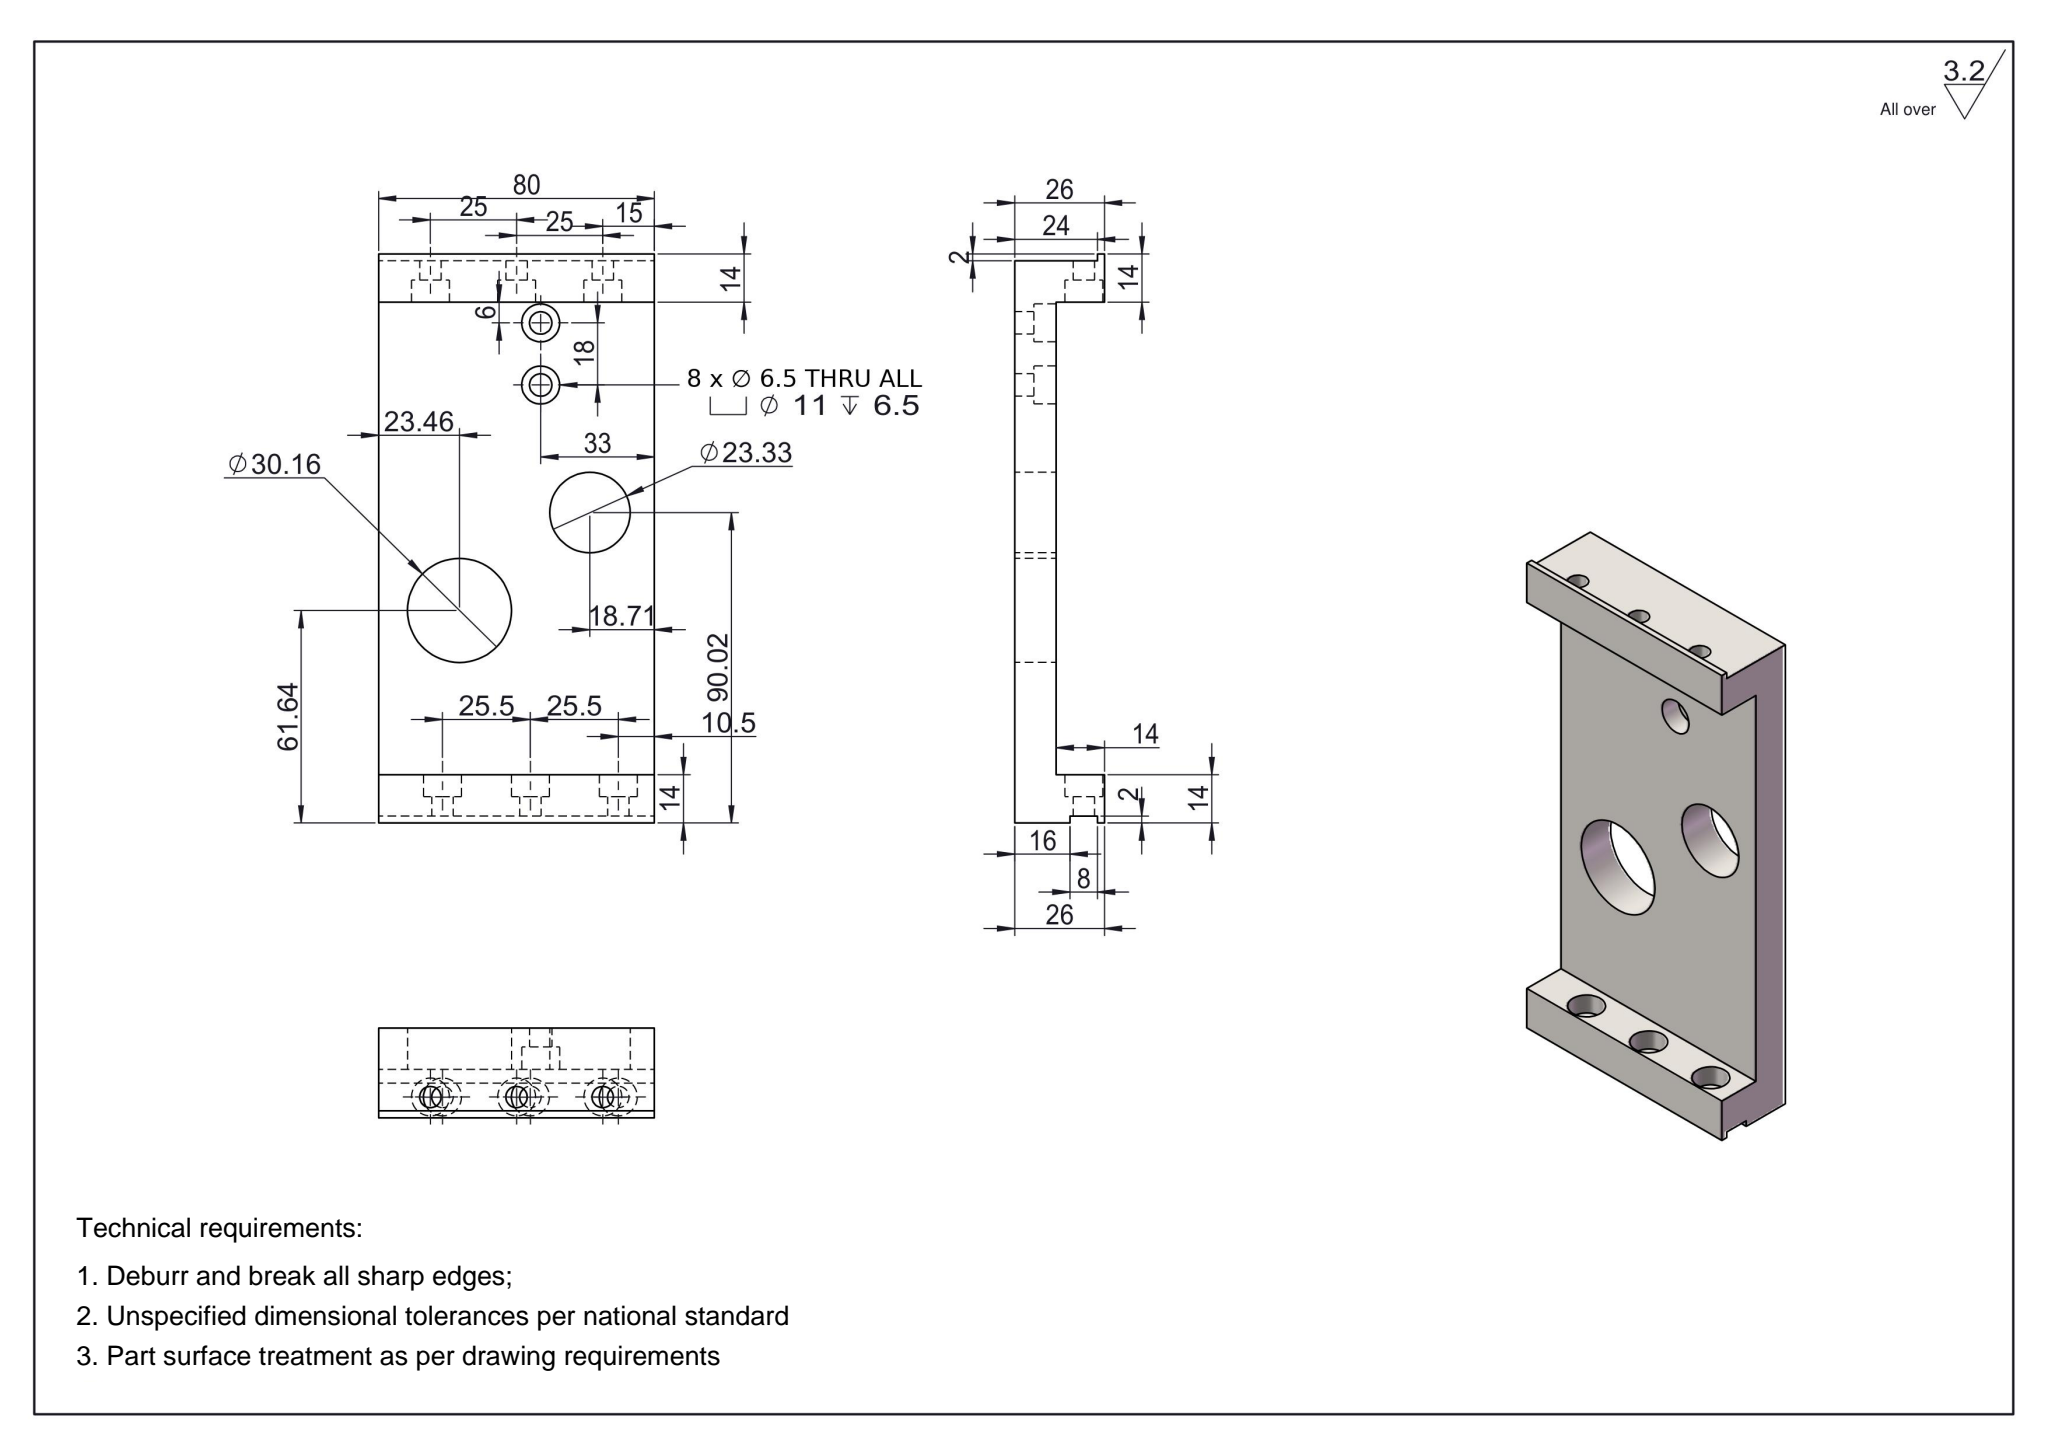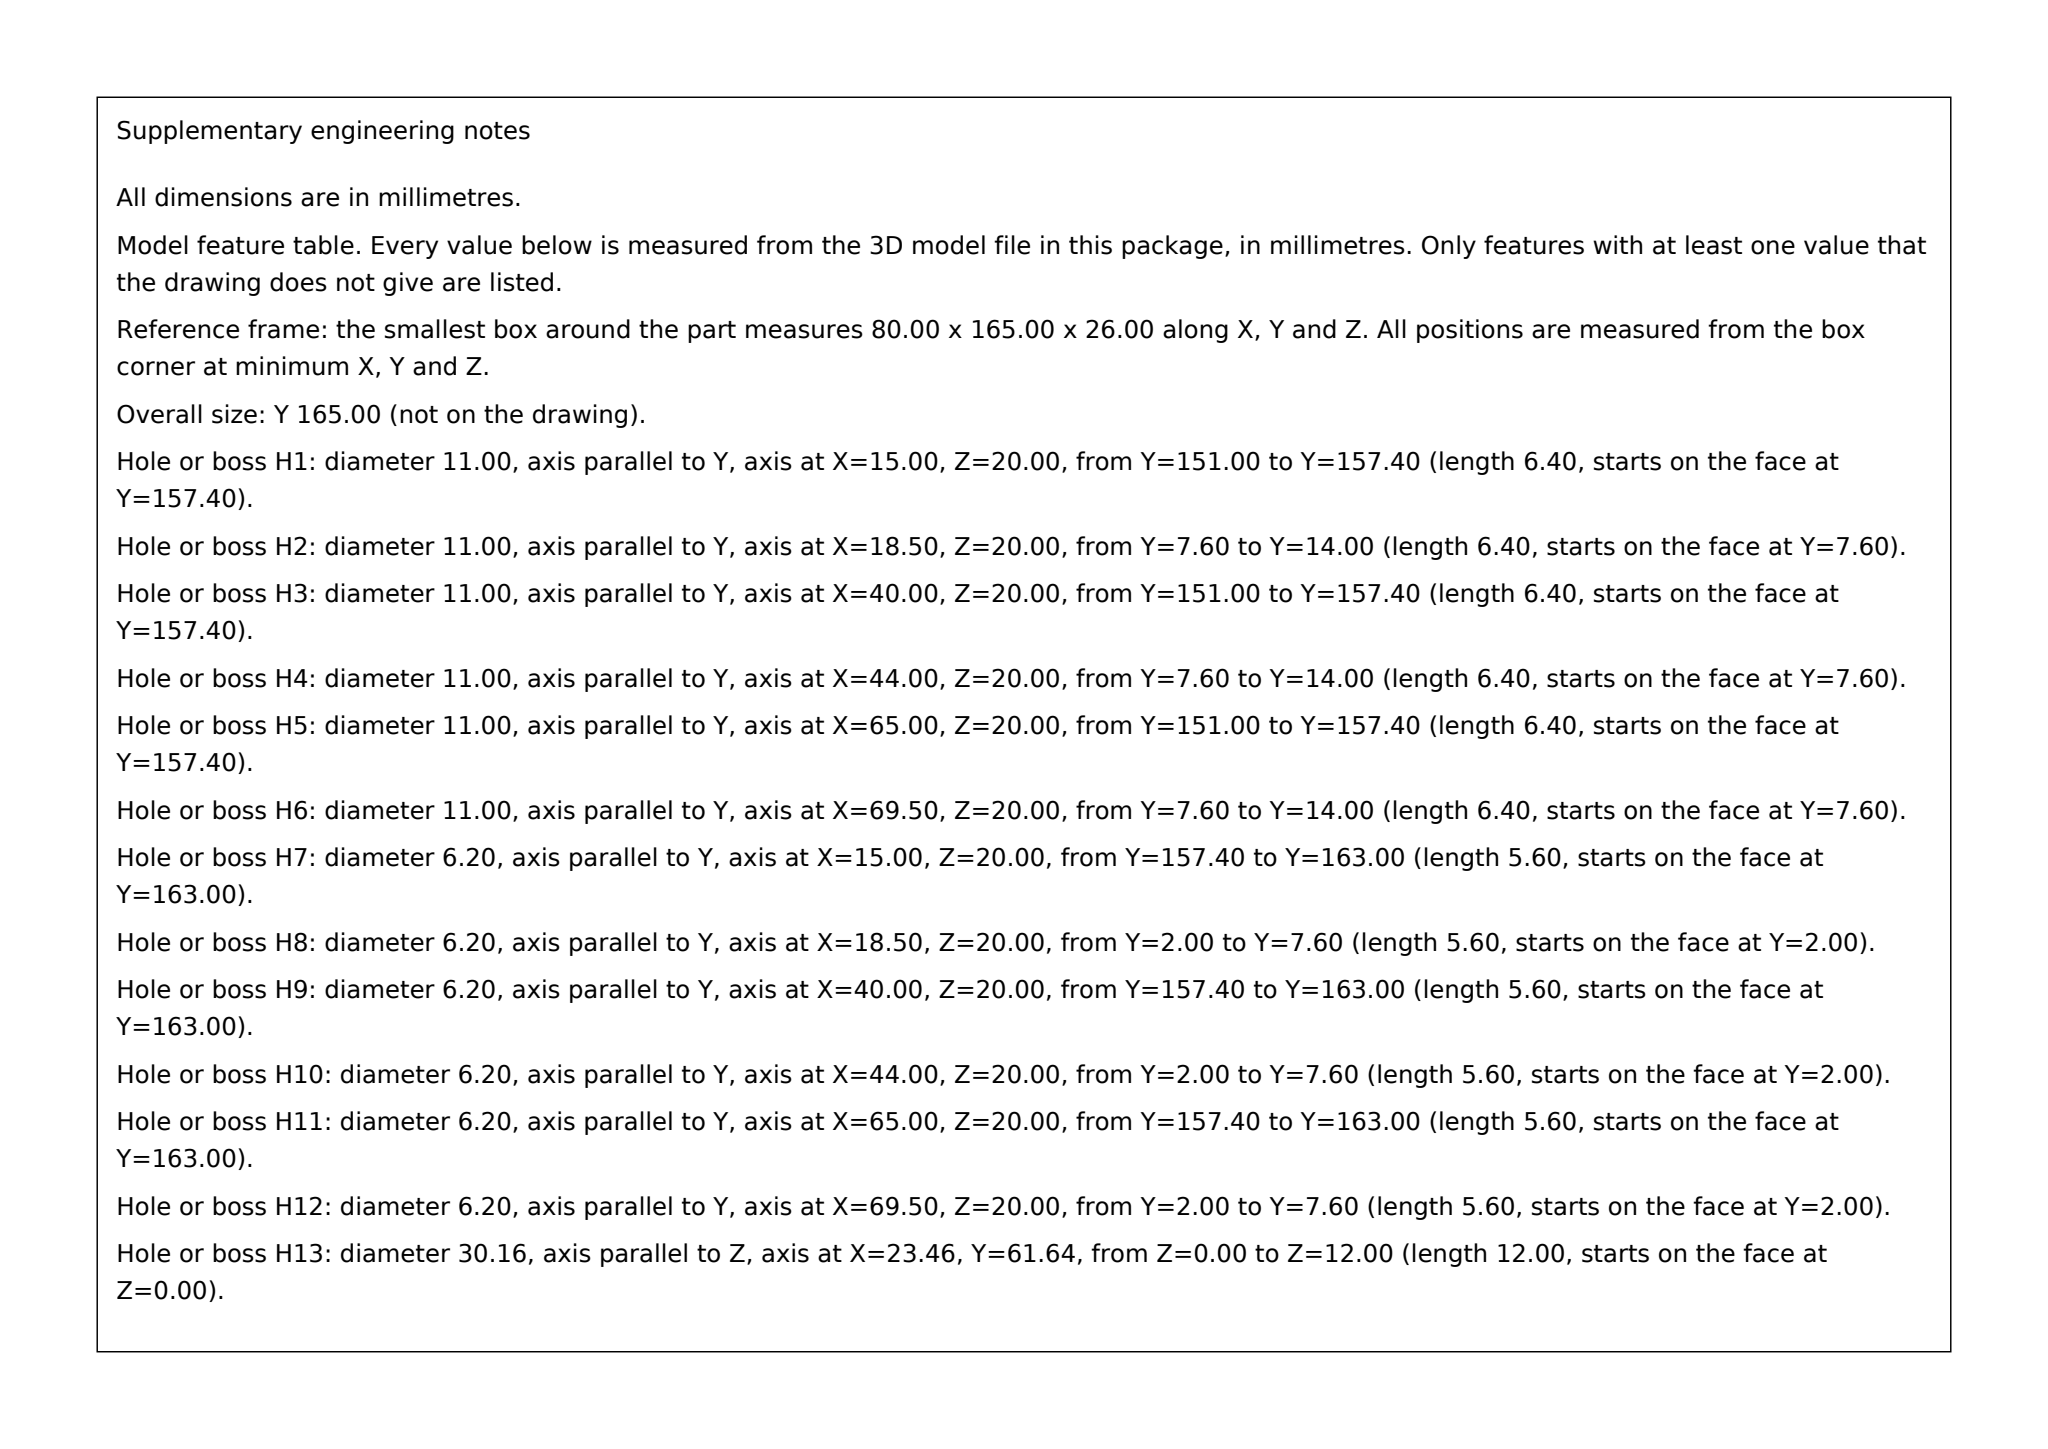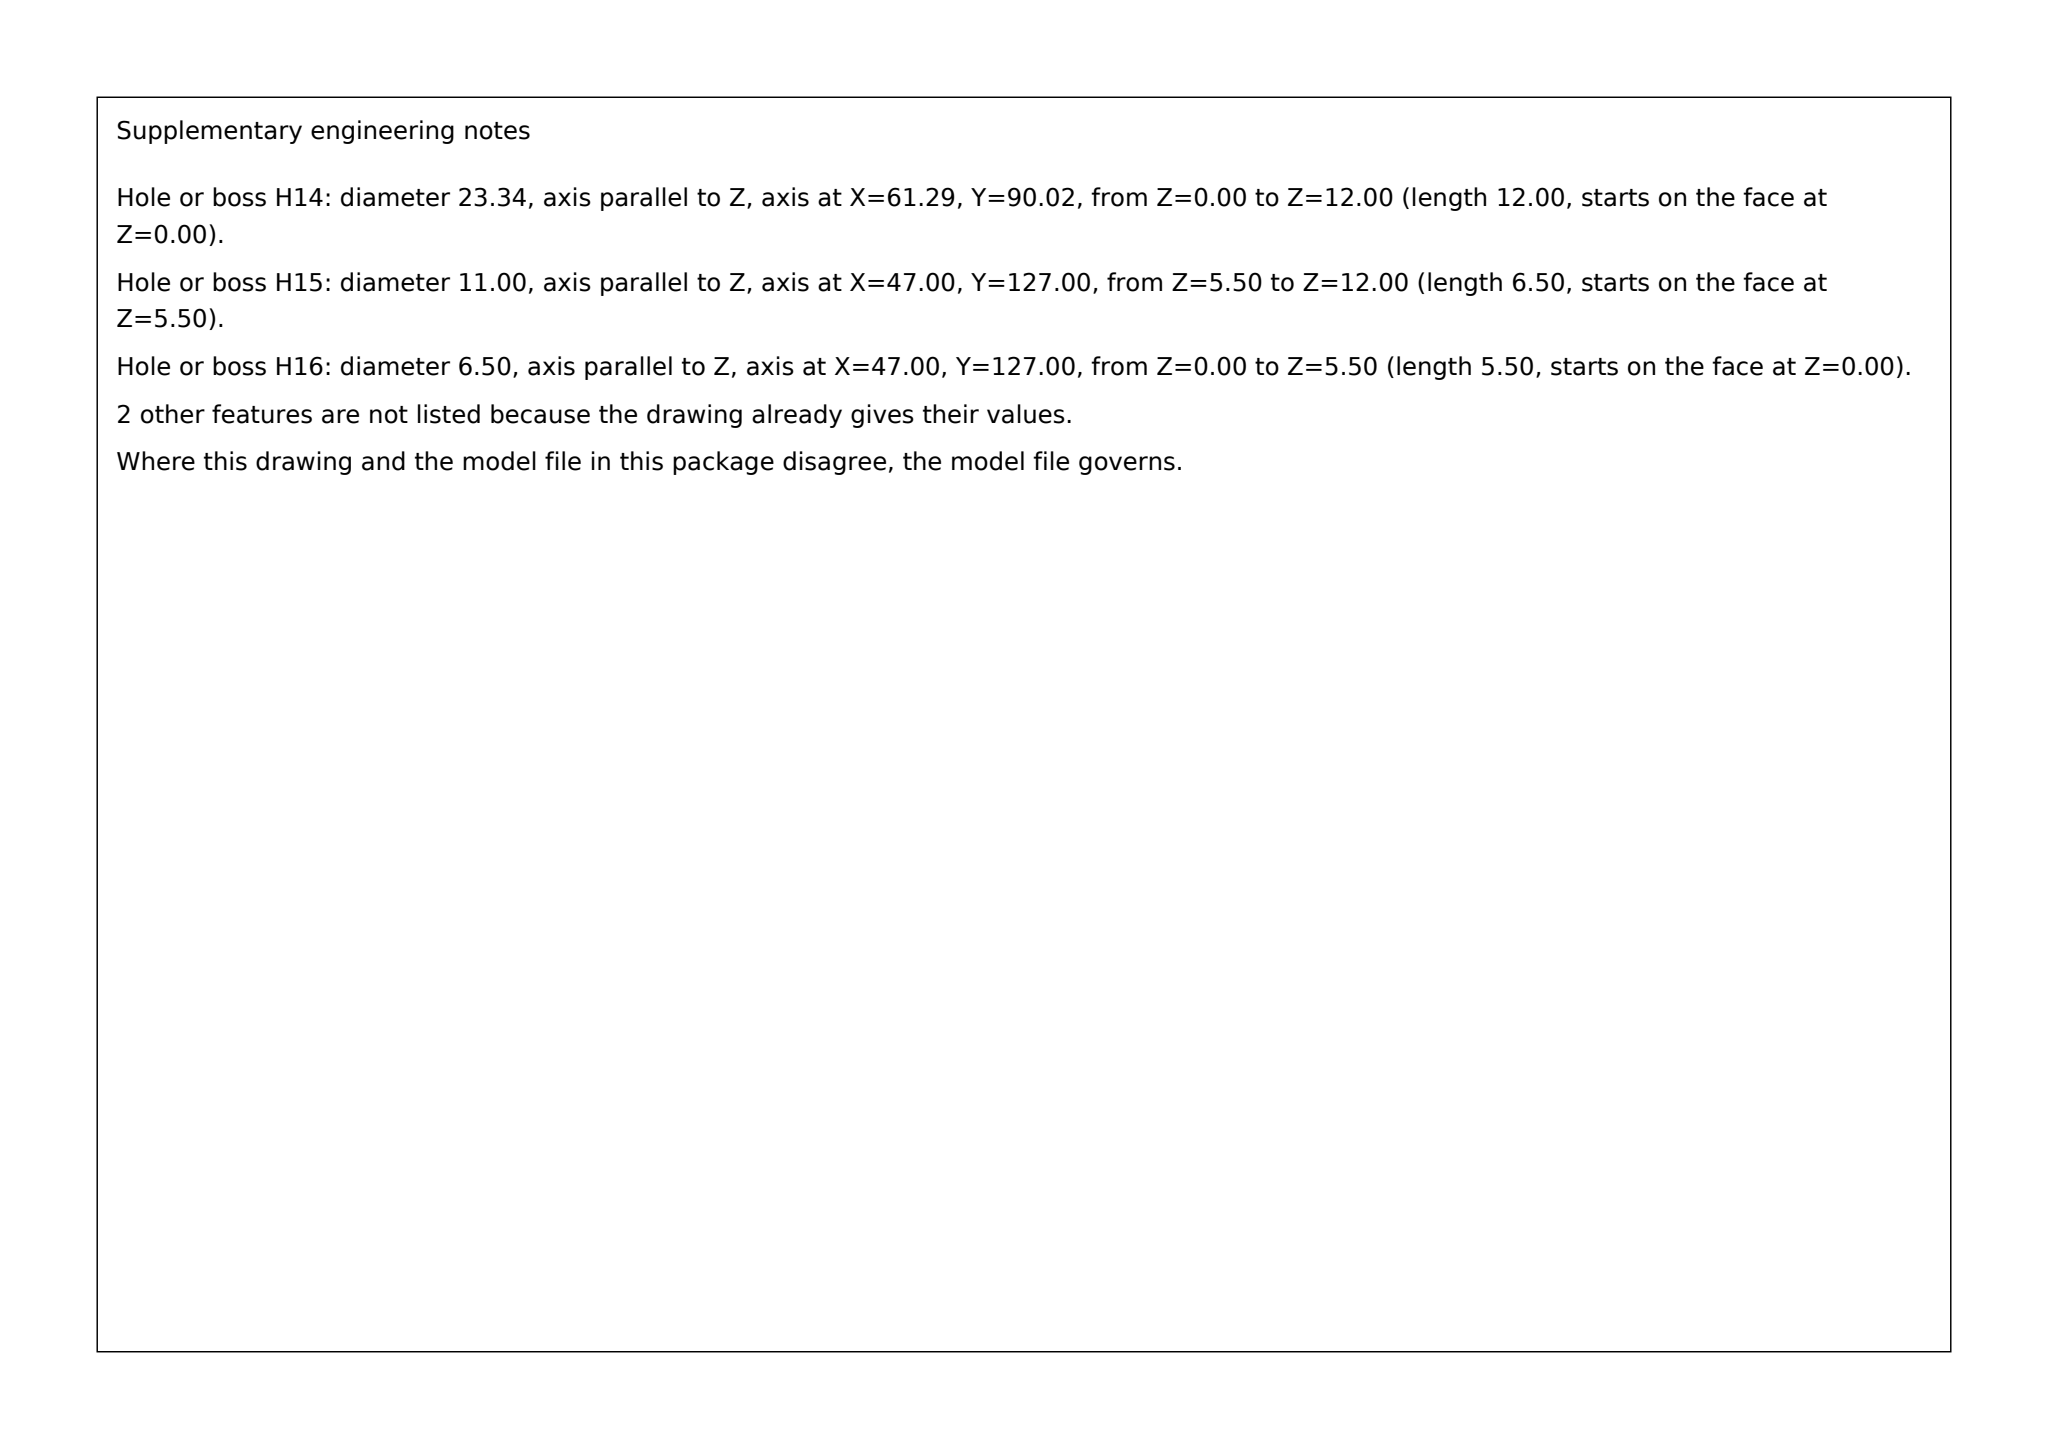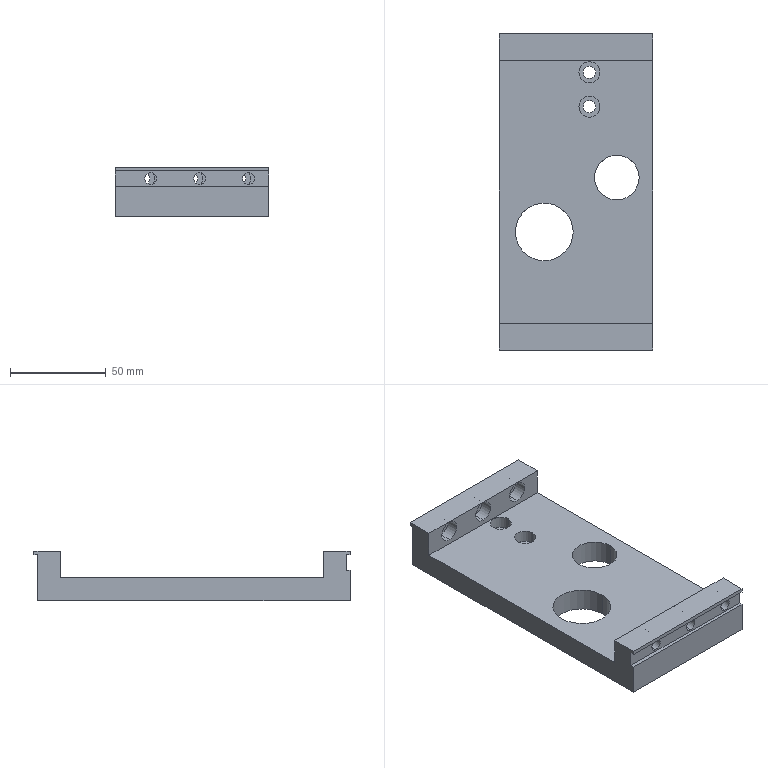Part | SolidWorks | mm | 1 solid | 60 faces | box 80 x 165 x 26 mm | volume 164671 mm3 | cylinder 36 | plane 24 | commonest cylinder face diameters 11 x16 6.2 x12 6.5 x4 30.161 x2 23.334 x2